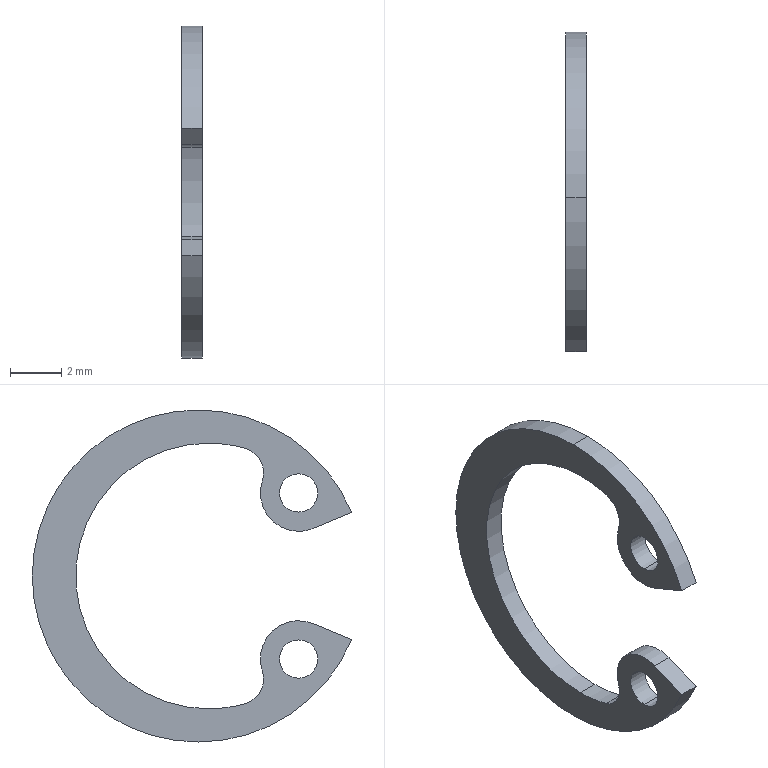Component | SolidWorks | UpperHousingAssembly-1_circlips for holes--type a gb-1 | 1 solid | 19 faces | box 0.8 x 12.51 x 13 mm | volume 40 mm3 | cylinder 15 | plane 4 | commonest cylinder face diameters 1.5 x4 3 x3 10.4 x3 13 x3 2 x2
build123d program:
from build123d import *

# Parameters (mm, degrees)
SKETCH1_R  = 0.75
BODY_DEPTH = 0.8


with BuildPart() as part:
    # Sketch1 → Body (new body)
    with BuildSketch(Plane.XY):
        with BuildLine():
            Line((1.865, -4.503), (2.487, -6.005))
            ThreePointArc((2.487, -6.005), (0, 6.5), (-2.487, -6.005))
            Line((-2.487, -6.005), (-1.865, -4.503))
            ThreePointArc((-1.865, -4.503), (-2.153, -2.908), (-3.723, -2.506))
            ThreePointArc((-3.723, -2.506), (-4.505, -2.441), (-4.999, -1.832))
            ThreePointArc((-4.999, -1.832), (0, 4.8), (4.999, -1.832))
            ThreePointArc((4.999, -1.832), (4.505, -2.441), (3.723, -2.506))
            ThreePointArc((3.723, -2.506), (2.153, -2.908), (1.865, -4.503))
        make_face()
        with Locations(Location((3.251, -3.929, 0), (0, 0, 180))):
            Circle(SKETCH1_R, mode=Mode.SUBTRACT)
        with Locations((-3.251, -3.929)):
            Circle(SKETCH1_R, mode=Mode.SUBTRACT)
    extrude(amount=-BODY_DEPTH)


solid = part.part

# Placed as in the assembly
solid = solid.moved(Location((1031.88, 1408.591, 1694.217), (0, 90, 0)))